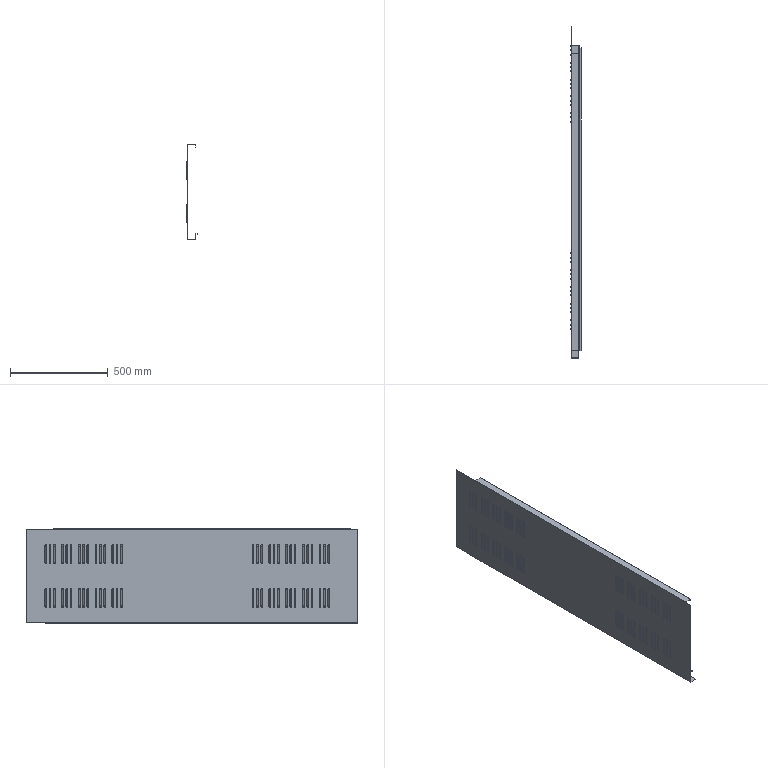Component | SolidWorks | AirFurnaceElectricalCabinet-LeftSidePlate-1 | 1 solid | 893 faces | volume 1227518 mm3 | cylinder 250 | torus 240 | sphere 240 | plane 163 | commonest cylinder face diameters 10 x120 7.6 x60 12.4 x60 3.9 x5 1.5 x5